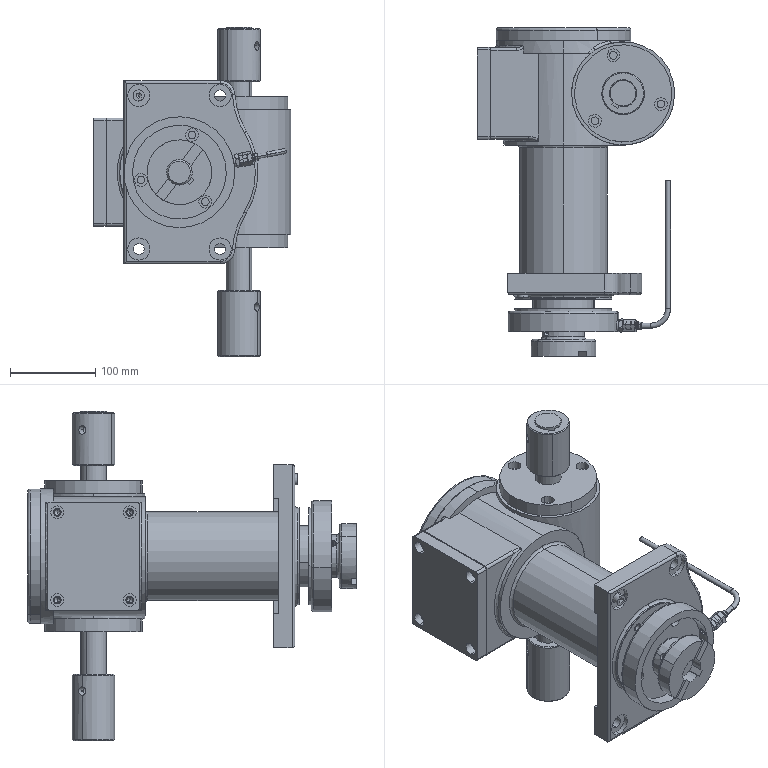Assembly | SolidWorks | mm | 28 component files | 28 solids | 1119 faces | box 231.5 x 385.4 x 386.5 mm | volume 4568033 mm3 | cylinder 471 | plane 259 | cone 230 | torus 147 | spline 12 | commonest cylinder face diameters 9 x60 6.8 x40 15 x38 66.641 x34 90 x34 6 x27 10 x20 30 x17
Bill of materials:
10 | 1 |  | Thin flat annular ring with a large central opening and three small through-holes equally spaced around the outer band.
1 | 1 |  | Slender solid round rod with a long straight section and a bend near one end. Its ends look rounded or domed.
11 | 1 |  | Screw-like shape: a cylindrical head with a hexagonal socket recess and a plain cylindrical shank with a chamfered tip.
12 | 1 |  | Ring-shaped part with an outer ring, an inner ring and a circle of rolling elements between them. The inner ring sticks out past the outer ring on one face.
13 | 1 |  | Stepped cylindrical shaft: a larger central section, shorter shoulder steps on each side, and smaller-diameter end journals with chamfered ends. Each end has a slot that looks like a keyway.
14 | 1 |  | Housing body with a rectangular mounting flange at one end, a cylindrical tubular section, and a cylindrical boss perpendicular to the tube's axis at the other end. It also has a block-shaped protrusion.
16 | 1 |  | Flat annular flange with a large central bore and three through-holes equally spaced. It has a rounded outer edge and a short raised spigot or step on one face.
17 | 1 |  | Thin flat rectangular plate with rounded corners, a large rectangular central cutout, and four corner through-holes.
18 | 1 |  | Toothed wheel with straight-sided rectangular teeth and a concave (throated) outer face, plus a cylindrical hub on one side. The bore has a keyway-like notch, and the hub has a radial hole.
19 | 1 |  | Thick rectangular plate with rounded corners, four corner through-holes, and a shallow rectangular pocket in one face.
20 | 1 |  | Small solid block with an obround profile: a rectangular body with fully rounded ends and slightly chamfered or rounded edges.
2 | 1 |  | Hexagonal prism, longer than it is wide across the flats, with a plain round through-hole along its axis.
21 | 1 |  | Short solid cylinder. One end has a straight slot cut across it; the other end narrows to a cone and finishes in a small flat face. Its shape resembles a slotted set screw, but no thread is modeled.
22 | 1 |  | Very thin, flat ring with a large central opening and three small through-holes spaced evenly around the ring. It looks like a gasket or shim.
227 | 2 |  | Round flange plate with a raised circular boss on one face. The boss has a counterbored recess leading to a smaller central through-bore, and three evenly spaced through-holes sit around the outer flange.
23 | 1 |  | Thin round disc or cover plate with three evenly spaced through-holes near the rim. One face has a shallow concentric circular feature, either a step or a recess, and the outer edges look slightly rounded.
24 | 1 |  | Tall cylindrical sleeve or collar. It has a central bore with a single keyway, a shallow counterbore or chamfer at the bore entrance, and one radial cross-hole through the wall. Both outer ends are chamfered.
25 | 1 |  | Plain solid cylindrical pin with chamfered or slightly rounded edges at both flat ends.
26 | 2 |  | Flat annular ring, like a washer or spacer, with a large central hole. The outer edge is chamfered on both faces.
28 | 1 |  | Long, slender stepped shaft. Near the middle is a larger-diameter section carrying helical thread-like or worm-like ridges, with stepped shoulders on either side. Each end journal has a small radial cross-hole.
29 | 1 |  | Short cylindrical collar with a central through-bore and one keyway. The bore entrance appears stepped or chamfered, there is one radial cross-hole through the wall, and both outer ends are chamfered.
3 | 1 |  | Flanged bushing: a hollow cylindrical sleeve with an outer flange at one end. The outside of the flange is chamfered toward the end face.
4 | 1 |  | Turned solid body made of several coaxial sections: a plain cylindrical shank, a hex-like section with chamfered corners, a reduced-diameter neck or groove, and a chamfered cylindrical collar at the end with a flat end face.
6 | 1 |  | Stepped hub: a large-diameter flange body with a smaller coaxial boss. It has a central bore with one keyway, a radial hole through the boss, rectangular notches or slots in the flange, and filleted outer edges.
8 | 1 |  | Short solid cylindrical pin. One end is flat and has a straight slot cut across its full diameter, with a small chamfer at the edge. The other end tapers to a cone that ends in a small flat tip. The shape looks like a slotted cone-point set-screw blank.
9 | 1 |  | Round, disc-shaped flange. One face has stepped bosses: a thin, slightly smaller step, then a smaller, taller cylindrical boss. A large through bore runs down the center. Three smaller through holes sit on a ring around it, evenly spaced. One small radial hole goes into the outer rim. The other face looks like it has a shallow recess with a raised outer lip.
Mates:
1. concentric | 6-1 face at (0, -313.2, 0) dir (0, -1, 0) r 25 | 9-1 face at (0, -302.2, 0) dir (0, -1, 0) r 65
2. concentric | 1-1 face at (80.401, -319.2, 16.115) dir (0.9805, 0, 0.1965) r 3 | 9-1 face at (63.732, -319.2, 12.774) dir (0.9805, 0, 0.1965) r 4.25
3. concentric | 14-1 face at (0, -288, 0) dir (0, 1, 0) r 52 | 13-1 face at (0, -281.2, 0) dir (0, -1, 0) r 15
4. concentric | 13-1 face at (0, -281.2, 0) dir (0, -1, 0) r 15 | 9-1 face at (0, -302.2, 0) dir (0, -1, 0) r 65
5. concentric | 13-1 face at (0, -281.2, 0) dir (0, -1, 0) r 15 | 6-1 face at (0, -313.2, 0) dir (0, -1, 0) r 25
6. concentric | 13-1 face at (-11.907, -327.2, 9.122) dir (0.7938, 0, -0.6082) r 785.398 | 6-1 face at (-19.845, -327.2, 15.204) dir (-0.7938, 0, 0.6082) r 4
7. concentric | 13-1 face at (0, -15.2, 0) dir (0, -1, 0) r 14 | 18-1 face at (0, -23.7, 0) dir (0, -1, 0) r 27
8. concentric | 14-1 face at (70, -47, -344) dir (0, 0, 1) r 36 | 28-1 face at (70, -47, -179.94) dir (0, 0, -1) r 15
9. concentric | 14-1 edge at (-85, -89.5, -51.5) dir (-1, 0, 0) r 3.4 | 17-1 edge at (-86, -89.5, -51.5) dir (1, 0, 0) r 4.5
10. concentric | 14-1 edge at (-85, -89.5, 51.5) dir (-1, 0, 0) r 3.4 | 17-1 edge at (-86, -89.5, 51.5) dir (1, 0, 0) r 4.5
11. concentric | 17-1 edge at (-86, -89.5, -51.5) dir (1, 0, 0) r 4.5 | 19-1 edge at (-101, -89.5, -51.5) dir (-1, 0, 0) r 7.5
12. concentric | 17-1 edge at (-86, -89.5, 51.5) dir (1, 0, 0) r 4.5 | 19-1 edge at (-101, -89.5, 51.5) dir (-1, 0, 0) r 7.5
13. concentric | 14-1 face at (0, 15, 0) dir (0, -1, 0) r 79 | 23-1 face at (0, 15.2, 0) dir (0, 1, 0) r 79
14. concentric | 14-1 edge at (34, 15, 58.89) dir (0, 1, 0) r 3.4 | 23-1 edge at (34, 30.2, 58.89) dir (0, 1, 0) r 7.5
15. concentric | 14-1 face at (0, 15, 0) dir (0, -1, 0) r 79 | 22-1 edge at (0, 15, 0) dir (0, 1, 0) r 58
16. concentric | 22-1 edge at (34, 15.2, 58.89) dir (0, 1, 0) r 4.5 | 23-1 edge at (34, 30.2, 58.89) dir (0, 1, 0) r 7.5
17. concentric | 227-1 edge at (70, -47, -88.5) dir (0, 0, 1) r 15.5 | 26-1 edge at (70, -47, -86.559) dir (0, 0, 1) r 15
18. coincident | 227-1 face at (70, -47, -85.7) dir (0, 0, -1) r 1448.623 | 26-1 face at (70, -47, -86.559) dir (0, 0, -1) r 1448.623
19. concentric | 24-1 face at (70, -47, -216.44) dir (0, 0, 1) r 25 | 28-1 face at (70, -47, -179.94) dir (0, 0, -1) r 15
20. concentric | 24-1 face at (108.469, -71.156, -157.94) dir (-0.8469, 0.5318, 0) r 5 | 28-1 face at (11.23, -10.097, -157.94) dir (0.8469, -0.5318, 0) r 5
21. concentric | 28-1 face at (70, -47, -179.94) dir (0, 0, -1) r 15 | 29-1 face at (70, -47, 106.06) dir (0, 0, 1) r 25
22. concentric | 28-1 face at (15.369, -12.695, 148.06) dir (0.8469, -0.5318, 0) r 5 | 29-1 face at (43.747, -30.515, 148.06) dir (0.8469, -0.5318, 0) r 5
23. concentric | 14-1 edge at (0, -288, 0) dir (0, -1, 0) r 57 | 10-1 edge at (0, -288.2, 0) dir (0, 1, 0) r 36
24. concentric | 14-1 edge at (46, -288, 0) dir (0, -1, 0) r 3.4 | 10-1 edge at (46, -288.2, 0) dir (0, 1, 0) r 4.5
25. concentric | 24-1 face at (108.469, -71.156, -157.94) dir (-0.8469, 0.5318, 0) r 5 | 25-1 face at (42.92, -29.995, -157.94) dir (-0.8469, 0.5318, 0) r 0.5
26. coincident | 18-1 face at (16.166, -119.7, -7.346) dir (-0.7938, 0, 0.6082) | 20-1 face at (13.733, -46.7, -10.521) dir (0.7938, 0, -0.6082)
27. coincident | 18-1 face at (11.3, -119.7, -13.696) dir (0.6082, 0, 0.7938) | 20-1 face at (12.821, -46.7, -11.712) dir (-0.6082, 0, -0.7938)
28. parallel | 13-1 face at (1.52, -343.2, 1.985) dir (-0.6082, 0, -0.7938) | 18-1 face at (16.166, -119.7, -7.346) dir (-0.6082, 0, -0.7938)
29. concentric | 13-1 face at (11.113, -27.7, -8.514) dir (0.7938, 0, -0.6082) r 2.5 | 20-1 face at (13.733, -46.7, -10.521) dir (-0.7938, 0, 0.6082) r 1.5
30. concentric | 2-1 face at (70.596, -319.2, 14.15) dir (-0.9805, 0, -0.1965) r 6.5 | 4-1 face at (80.401, -319.2, 16.115) dir (-0.9805, 0, -0.1965) r 6.5
31. coincident | 2-1 edge at (80.401, -319.2, 16.115) dir (-0.9805, 0, -0.1965) r 6.5 | 4-1 face at (80.401, -319.2, 16.115) dir (0.9805, 0, 0.1965)
32. coincident | 1-1 face at (80.401, -319.2, 16.115) dir (-0.9805, 0, -0.1965) | 4-1 face at (80.401, -319.2, 16.115) dir (0.9805, 0, 0.1965)
33. tangent | 4-1 face at (63.732, -319.2, 12.774) dir (-0.9805, 0, -0.1965) | 9-1 face at (0, -302.2, 0) dir (0, -1, 0) r 65
34. coincident | 14-1 face at (0, -288, 0) dir (0, -1, 0) | 10-1 face at (0, -288, 0) dir (0, 1, 0)
35. concentric | 16-1 face at (0, -85, 0) dir (0, 1, 0) r 52 | 23-1 face at (0, 15.2, 0) dir (0, 1, 0) r 79
36. concentric | 14-1 edge at (-21.5, -85, -37.239) dir (0, 1, 0) r 3.4 | 16-1 edge at (-21.5, -72, -37.239) dir (0, 1, 0) r 7.5
37. coincident | 14-1 face at (0, -85, 0) dir (0, 1, 0) | 16-1 face at (0, -85, 0) dir (0, -1, 0)
38. concentric | 14-1 face at (70, -47, 73.5) dir (0, 0, -1) r 60.5 | 227-1 face at (70, -47, -73.5) dir (0, 0, -1) r 57
39. concentric | 14-1 face at (-47.662, -278, 90) dir (0, -1, 0) r 13 | 11-1 face at (-47.662, -258, 90) dir (0, -1, 0) r 4.5
40. coincident | 14-1 face at (-47.662, -278, 90) dir (0, -1, 0) | 11-1 face at (-47.662, -278, 90) dir (0, 1, 0)
41. concentric | 1-1 face at (80.401, -319.2, 16.115) dir (0.9805, 0, 0.1965) r 3 | 3-1 edge at (84.813, -319.2, 16.999) dir (-0.9805, 0, -0.1965) r 3.5
42. coincident | 2-1 face at (84.813, -319.2, 16.999) dir (0.9805, 0, 0.1965) | 3-1 edge at (84.813, -319.2, 16.999) dir (-0.9805, 0, -0.1965) r 3.5
43. tangent | 6-1 face at (0, -313.2, 0) dir (0, -1, 0) r 25 | 8-1 face at (-20.196, -326.234, 14.747) dir (-0.7938, 0, 0.6082)
44. concentric | 18-1 face at (0, -30.7, 0) dir (0.7938, 0, -0.6082) r 3.4 | 21-1 face at (-11.907, -30.7, 9.122) dir (0.7938, 0, -0.6082) r 2.923
45. tangent | 18-1 face at (0, -23.7, 0) dir (0, -1, 0) r 27 | 21-1 face at (-21.433, -30.7, 16.42) dir (-0.7938, 0, 0.6082)
46. coincident | 14-1 face at (-85, 0, 0) dir (-1, 0, 0) | 17-1 face at (-85, 1.5, -58.5) dir (1, 0, 0)
47. coincident | 17-1 face at (-86, 1.5, -58.5) dir (-1, 0, 0) | 19-1 face at (-86, -47, 0) dir (1, 0, 0)
48. coincident | 14-1 face at (0, 15, 0) dir (0, 1, 0) | 22-1 face at (0, 15, 0) dir (0, -1, 0)
49. coincident | 22-1 face at (0, 15.2, 0) dir (0, 1, 0) | 23-1 face at (0, 15.2, 0) dir (0, -1, 0)
50. coincident | 6-1 face at (0, -313.2, 0) dir (0, 1, 0) | 9-1 face at (0, -313.2, 0) dir (0, -1, 0)
51. coincident | 10-1 face at (0, -288.2, 0) dir (0, -1, 0) | 9-1 edge at (0, -288.2, 0) dir (0, 1, 0) r 36
52. coincident | 14-1 face at (70, -47, -73.5) dir (0, 0, -1) | 227-1 face at (70, -47, -73.5) dir (0, 0, 1)
53. parallel | 14-1 face at (0, -258, 0) dir (0, 1, 0) | 1-1 face at (122.562, -149.2, 24.565) dir (0, 1, 0)
54. concentric | 6-1 face at (-19.845, -327.2, 15.204) dir (-0.7938, 0, 0.6082) r 4 | 8-1 face at (-7.938, -327.2, 6.082) dir (-0.7938, 0, 0.6082) r 3.75
55. concentric | 12-1 face at (0, -287.803, 0) dir (0, 1, 0) r 36 | 13-1 face at (0, -281.2, 0) dir (0, -1, 0) r 15